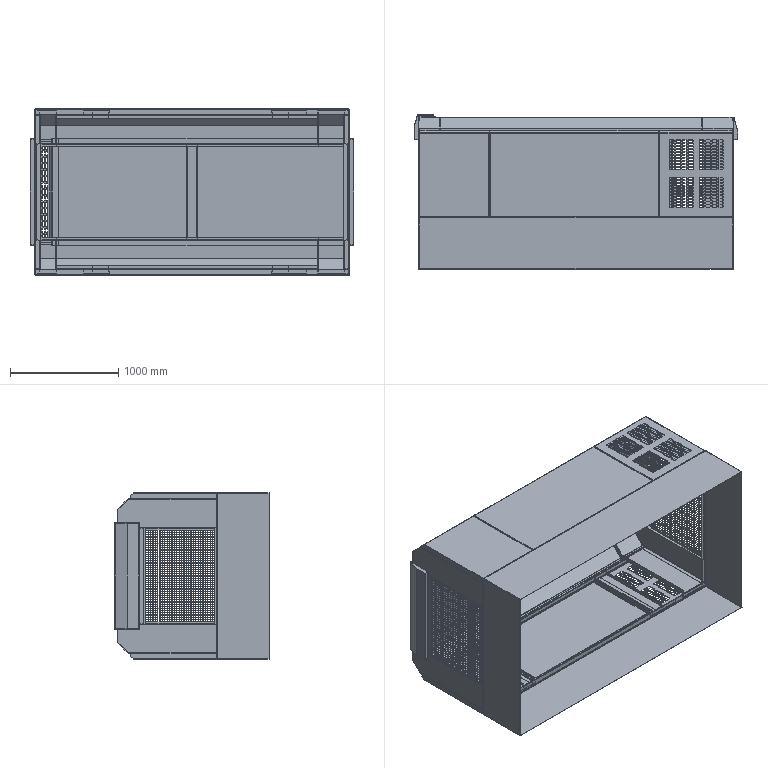Assembly | NX | mm | 23 component files | 183 solids | 3586 faces | box 2990 x 1422 x 1540 mm | volume 39840692 mm3 | plane 2236 | cylinder 1348 | spline 2 | commonest cylinder face diameters 20 x760 2 x202 6 x175 10 x171 4 x32 7 x8
Bill of materials:
unnamed part 1 | 2 |  | Shallow rectangular tray-like panel that looks like sheet metal. It has four rectangular fields of rounded-end slots, with folded edge flanges and a recessed strip along one edge.
unnamed part 2 | 1 |  | Open rectangular frame or sleeve made of thin walls that looks like sheet metal. It is a four-sided band with no front or back face.
unnamed part 3 | 2 |  | Flat rectangular panel with shallow folded flanges along its long edges, like a plain shelf or cover plate.
unnamed part 4 | 1 |  | Box-like formed sheet part with a flat top, a deep side wall, and small flanged ends. The side profile has a chamfered corner.
unnamed part 5 | 4 |  | Long, narrow, flat tray or channel that looks like sheet metal, with low upturned flanges along both long sides. The flanges at the two ends point in opposite directions (a joggled or Z-type end condition).
unnamed part 6 | 1 |  | Tall, narrow bent sheet profile. Its outline is tapered (trapezoidal), with a top flange and a stepped offset bottom flange.
unnamed part 7 | 1 |  | Long straight profile with a constant cross-section. The section has a horizontal leg, a 45-degree angled segment, a vertical leg, and small return lips at both ends.
unnamed part 8 | 2 |  | Flat rectangular panel made of a square-grid mesh inside a thin perimeter frame.
unnamed part 9 | 1 |  | Open channel or trough made of formed sheet. It has a base, a tall side wall, and an end wall with a chamfered (angled) lower corner and small flanges.
unnamed part 10 | 1 |  | Open trough of formed sheet with a flat base, a tall back wall, and a closed end wall with an angled chamfer between base and wall. It has small flanges at the open end.
unnamed part 11 | 1 |  | Long straight profile with a constant cross-section. The section has a horizontal leg, a 45-degree angled segment, a vertical leg, and small return lips at the ends.
unnamed part 12 | 2 |  | Shallow rectangular tray-like panel of formed sheet with a plain flat face, folded edge flanges, and a recessed lip along one edge. It looks like unnamed part 1 but has no slot pattern.
unnamed part 13 | 1 |  | Flat thin rectangular plate or sheet with no visible holes, bends, or cut-outs.
unnamed part 14 | 1 |  | Elongated sheet-metal style formed cover, open on one side like a channel, with folded flanges along its length and folded return walls at both ends. One end corner is chamfered in profile.
unnamed part 15 | 1 |  | Long straight post or column with an open channel-type cross-section, capped at each end by a flat rectangular plate with rounded corners and two through holes.
unnamed part 16 | 1 |  | Tall sheet-metal style bent corner panel with two main walls at an angle. One wall has a perforated grid of elongated slots (about 4 columns by 15 rows). It also has narrow folded edge flanges, and the plan profile includes an angled segment.
Mates:
1. touch align | side_column_rear_right 1 face | bottom_beam 1 face
2. touch align | side_column_rear_right 1 face | bottom_beam 1 face
3. touch align | side_column_rear_left 1 face | bottom_beam 1 face
4. touch align | side_column_rear_left 1 face | bottom_beam 1 face
5. touch align | side_column_front_right 1 face | bottom_beam 1 face
6. touch align | side_column_front_right 1 face | bottom_beam 1 face
7. touch align | side_column_front_left 1 face | bottom_beam 1 face
8. touch align | side_column_front_left 1 face | bottom_beam 1 face
9. touch align | upper_right_crossbeam 1 face | side_column_rear_right 1 face
10. touch align | upper_right_crossbeam 1 face | side_column_front_right 1 face
11. touch align | upper_right_crossbeam 1 face | side_column_front_right 1 face
12. touch align | upper_left_crossbeam 1 face | side_column_rear_left 1 face
13. touch align | upper_left_crossbeam 1 face | side_column_rear_left 1 face
14. touch align | upper_left_crossbeam 1 face | side_column_rear_left 1 face
15. touch align | side_cover_plate_rear_left 2 face | side_column_rear_left 1 face
16. touch align | side_cover_plate_rear_left 2 face | side_column_rear_left 1 face
17. touch align | side_cover_plate_rear_left 2 face | bottom_beam 1 face
18. touch align | side_cover_plate_rear_left 1 face | side_column_rear_right 1 face
19. touch align | side_cover_plate_rear_left 1 face | side_column_rear_right 1 face
20. touch align | side_cover_plate_rear_left 1 face | bottom_beam 1 face
21. touch align | side_cover_plate_front_left 2 face | side_column_front_left 1 face
22. touch align | side_cover_plate_front_left 2 face | side_column_front_left 1 face
23. touch align | side_cover_plate_front_left 2 face | bottom_beam 1 face
24. touch align | side_cover_plate_front_left 1 face | side_column_front_right 1 face
25. touch align | side_cover_plate_front_left 1 face | side_column_front_right 1 face
26. touch align | side_cover_plate_front_left 1 face | bottom_beam 1 face
27. touch align | side_column_rear_right 1 face | bottom_beam 1 face
28. touch align | side_column_rear_left 1 face | bottom_beam 1 face
29. touch align | side_column_front_right 1 face | bottom_beam 1 face
30. touch align | side_column_front_left 1 face | bottom_beam 1 face
31. touch align | column_left_front 4 face | upper_left_crossbeam 1 face
32. touch align | column_left_front 4 face | upper_left_crossbeam 1 face
33. distance | column_left_front 4 face | side_cover_plate_rear_left 2 face
34. touch align | column_left_front 3 face | upper_right_crossbeam 1 face
35. touch align | column_left_front 3 face | upper_right_crossbeam 1 face
36. distance | column_left_front 3 face | side_cover_plate_rear_left 1 face
37. touch align | column_left_front 2 face | upper_left_crossbeam 1 face
38. touch align | column_left_front 2 face | upper_left_crossbeam 1 face
39. distance | column_left_front 2 face | side_cover_plate_front_left 2 face
40. touch align | column_left_front 1 face | upper_right_crossbeam 1 face
41. touch align | column_left_front 1 face | upper_right_crossbeam 1 face
42. distance | column_left_front 1 face | side_cover_plate_front_left 1 face
43. touch align | door 2 face | upper_right_crossbeam 1 face
44. touch align | door 2 face | bottom_beam 1 face
45. distance | door 2 face | side_cover_plate_front_left 1 face
46. touch align | door 1 face | upper_left_crossbeam 1 face
47. touch align | door 1 face | bottom_beam 1 face
48. distance | door 1 face | side_cover_plate_front_left 2 face
49. touch align | top_beam 1 face | upper_right_crossbeam 1 face
50. touch align | top_beam 1 face | upper_right_crossbeam 1 face
51. center | front_rear_baffle 2 face | front_rear_baffle 2 face | side_column_rear_right 1 face | side_column_rear_left 1 face
52. touch align | front_rear_baffle 2 face | side_column_rear_right 1 face
53. center | front_rear_baffle 1 face | front_rear_baffle 1 face | side_column_front_right 1 face | side_column_front_left 1 face
54. touch align | front_rear_baffle 1 face | side_column_front_left 1 face
55. touch align | upper_beam_front 1 face | side_column_front_right 1 face
56. touch align | upper_beam_front 1 face | side_column_front_left 1 face
57. center | upper_beam_front 1 face | upper_beam_front 1 face | side_column_front_right 1 face | side_column_front_left 1 face
58. touch align | upper_beam_rear 1 face | side_column_rear_right 1 face
59. touch align | upper_beam_rear 1 face | side_column_rear_left 1 face
60. center | upper_beam_rear 1 face | upper_beam_rear 1 face | side_column_rear_left 1 face | side_column_rear_right 1 face
61. touch align | top_cover 1 face | upper_left_crossbeam 1 face
62. center | top_cover 1 face | top_cover 1 face | upper_beam_front 1 face | upper_beam_rear 1 face
63. touch align | top_cover 1 face | upper_beam_front 1 face